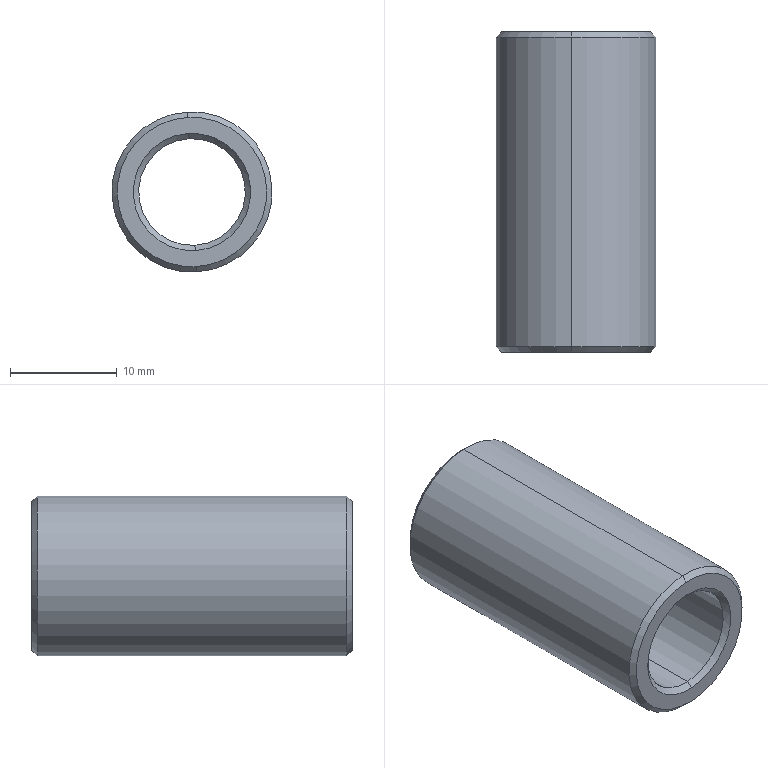Component | SolidWorks | JB_T8013.1-1999LocatingBushingA18-3 | 1 solid | 14 faces | box 15 x 30 x 15 mm | volume 2923 mm3 | cone 6 | cylinder 4 | torus 2 | plane 2 | commonest cylinder face diameters 10 x2 15 x2 | material Nickel
build123d program:
from build123d import *

# Parameters (mm, degrees)
SKETCH1_R          = 7.5
SKETCH1_R_2        = 5
BASE_EXTRUDE_DEPTH = 30
FILLET1_R          = 1
CHAMFER1_SIZE      = 0.5


with BuildPart() as part:
    # Sketch1 → Base-Extrude (new body)
    with BuildSketch(Plane.XY):
        Circle(SKETCH1_R)
        Circle(SKETCH1_R_2, mode=Mode.SUBTRACT)
    extrude(amount=-BASE_EXTRUDE_DEPTH)

    # Fillet1
    fillet1_edges = [part.edges().sort_by_distance(p)[0] for p in [
        (-5, 0, 0),
    ]]
    fillet(fillet1_edges, radius=FILLET1_R)

    # Chamfer1
    chamfer1_edges = [part.edges().sort_by_distance(p)[0] for p in [
        (-7.5, 0, 0),
        (-7.5, 0, -30),
        (-5, 0, -30),
    ]]
    chamfer(chamfer1_edges, length=CHAMFER1_SIZE)


solid = part.part

# Placed as in the assembly
solid = solid.moved(Location((45.466, 305, -26.25), (-90, 0, 0)))
STEP:
#1=COLOUR_RGB('',0.7922,0.8196,0.9333);
#2=FILL_AREA_STYLE_COLOUR('',#1);
#3=FILL_AREA_STYLE('',(#2));
#4=SURFACE_STYLE_FILL_AREA(#3);
#5=SURFACE_SIDE_STYLE('',(#4));
#6=SURFACE_STYLE_USAGE(.BOTH.,#5);
#7=PRESENTATION_STYLE_ASSIGNMENT((#6));
#8=CARTESIAN_POINT('',(1.775,12.008,-0.7583));
#9=VERTEX_POINT('',#8);
#10=CARTESIAN_POINT('',(1.805,12.008,-1.309));
#11=VERTEX_POINT('',#10);
#12=CARTESIAN_POINT('',(1.79,12.008,-1.033));
#13=DIRECTION('',(0.,1.,0.));
#14=DIRECTION('',(-0.05508,0.,0.9985));
#15=AXIS2_PLACEMENT_3D('',#12,#13,#14);
#16=CIRCLE('',#15,0.2756);
#17=EDGE_CURVE('',#9,#11,#16,.T.);
#18=ORIENTED_EDGE('',*,*,#17,.F.);
#19=CARTESIAN_POINT('',(1.774,11.988,-0.7386));
#20=VERTEX_POINT('',#19);
#21=CARTESIAN_POINT('',(1.775,12.008,-0.7583));
#22=DIRECTION('',(-0.03895,-0.7071,0.706));
#23=VECTOR('',#22,39.37);
#24=LINE('',#21,#23);
#25=EDGE_CURVE('',#9,#20,#24,.T.);
#26=ORIENTED_EDGE('',*,*,#25,.T.);
#27=CARTESIAN_POINT('',(1.806,11.988,-1.328));
#28=VERTEX_POINT('',#27);
#29=CARTESIAN_POINT('',(1.79,11.988,-1.033));
#30=DIRECTION('',(0.,-1.,0.));
#31=DIRECTION('',(-0.05508,0.,0.9985));
#32=AXIS2_PLACEMENT_3D('',#29,#30,#31);
#33=CIRCLE('',#32,0.2953);
#34=EDGE_CURVE('',#28,#20,#33,.T.);
#35=ORIENTED_EDGE('',*,*,#34,.F.);
#36=CARTESIAN_POINT('',(1.805,12.008,-1.309));
#37=DIRECTION('',(0.03895,-0.7071,-0.706));
#38=VECTOR('',#37,39.37);
#39=LINE('',#36,#38);
#40=EDGE_CURVE('',#11,#28,#39,.T.);
#41=ORIENTED_EDGE('',*,*,#40,.F.);
#42=EDGE_LOOP('',(#18,#26,#35,#41));
#43=FACE_OUTER_BOUND('',#42,.T.);
#44=CARTESIAN_POINT('',(1.79,12.008,-1.033));
#45=DIRECTION('',(0.,-1.,0.));
#46=DIRECTION('',(0.05508,0.,-0.9985));
#47=AXIS2_PLACEMENT_3D('',#44,#45,#46);
#48=CONICAL_SURFACE('',#47,0.2756,0.7854);
#49=ADVANCED_FACE('',(#43),#48,.T.);
#50=CARTESIAN_POINT('',(1.805,10.827,-1.309));
#51=VERTEX_POINT('',#50);
#52=CARTESIAN_POINT('',(1.775,10.827,-0.7583));
#53=VERTEX_POINT('',#52);
#54=CARTESIAN_POINT('',(1.79,10.827,-1.033));
#55=DIRECTION('',(0.,-1.,0.));
#56=DIRECTION('',(-0.05508,0.,0.9985));
#57=AXIS2_PLACEMENT_3D('',#54,#55,#56);
#58=CIRCLE('',#57,0.2756);
#59=EDGE_CURVE('',#51,#53,#58,.T.);
#60=ORIENTED_EDGE('',*,*,#59,.F.);
#61=CARTESIAN_POINT('',(1.806,10.846,-1.328));
#62=VERTEX_POINT('',#61);
#63=CARTESIAN_POINT('',(1.806,10.846,-1.328));
#64=DIRECTION('',(0.03895,0.7071,-0.706));
#65=VECTOR('',#64,39.37);
#66=LINE('',#63,#65);
#67=EDGE_CURVE('',#51,#62,#66,.T.);
#68=ORIENTED_EDGE('',*,*,#67,.T.);
#69=CARTESIAN_POINT('',(1.774,10.846,-0.7386));
#70=VERTEX_POINT('',#69);
#71=CARTESIAN_POINT('',(1.79,10.846,-1.033));
#72=DIRECTION('',(0.,1.,0.));
#73=DIRECTION('',(-0.05508,0.,0.9985));
#74=AXIS2_PLACEMENT_3D('',#71,#72,#73);
#75=CIRCLE('',#74,0.2953);
#76=EDGE_CURVE('',#70,#62,#75,.T.);
#77=ORIENTED_EDGE('',*,*,#76,.F.);
#78=CARTESIAN_POINT('',(1.774,10.846,-0.7386));
#79=DIRECTION('',(-0.03895,0.7071,0.706));
#80=VECTOR('',#79,39.37);
#81=LINE('',#78,#80);
#82=EDGE_CURVE('',#53,#70,#81,.T.);
#83=ORIENTED_EDGE('',*,*,#82,.F.);
#84=EDGE_LOOP('',(#60,#68,#77,#83));
#85=FACE_OUTER_BOUND('',#84,.T.);
#86=CARTESIAN_POINT('',(1.79,10.846,-1.033));
#87=DIRECTION('',(0.,1.,0.));
#88=DIRECTION('',(-0.05508,0.,0.9985));
#89=AXIS2_PLACEMENT_3D('',#86,#87,#88);
#90=CONICAL_SURFACE('',#89,0.2953,0.7854);
#91=ADVANCED_FACE('',(#85),#90,.T.);
#92=CARTESIAN_POINT('',(1.779,10.846,-0.8369));
#93=VERTEX_POINT('',#92);
#94=CARTESIAN_POINT('',(1.801,10.846,-1.23));
#95=VERTEX_POINT('',#94);
#96=CARTESIAN_POINT('',(1.79,10.846,-1.033));
#97=DIRECTION('',(0.,-1.,0.));
#98=DIRECTION('',(-0.05508,0.,0.9985));
#99=AXIS2_PLACEMENT_3D('',#96,#97,#98);
#100=CIRCLE('',#99,0.1969);
#101=EDGE_CURVE('',#93,#95,#100,.T.);
#102=ORIENTED_EDGE('',*,*,#101,.F.);
#103=CARTESIAN_POINT('',(1.778,10.827,-0.8173));
#104=VERTEX_POINT('',#103);
#105=CARTESIAN_POINT('',(1.778,10.827,-0.8173));
#106=DIRECTION('',(-0.03895,-0.7071,0.706));
#107=VECTOR('',#106,39.37);
#108=LINE('',#105,#107);
#109=EDGE_CURVE('',#93,#104,#108,.T.);
#110=ORIENTED_EDGE('',*,*,#109,.T.);
#111=CARTESIAN_POINT('',(1.802,10.827,-1.25));
#112=VERTEX_POINT('',#111);
#113=CARTESIAN_POINT('',(1.79,10.827,-1.033));
#114=DIRECTION('',(0.,1.,0.));
#115=DIRECTION('',(-0.05508,0.,0.9985));
#116=AXIS2_PLACEMENT_3D('',#113,#114,#115);
#117=CIRCLE('',#116,0.2165);
#118=EDGE_CURVE('',#112,#104,#117,.T.);
#119=ORIENTED_EDGE('',*,*,#118,.F.);
#120=CARTESIAN_POINT('',(1.802,10.827,-1.25));
#121=DIRECTION('',(0.03895,-0.7071,-0.706));
#122=VECTOR('',#121,39.37);
#123=LINE('',#120,#122);
#124=EDGE_CURVE('',#95,#112,#123,.T.);
#125=ORIENTED_EDGE('',*,*,#124,.F.);
#126=EDGE_LOOP('',(#102,#110,#119,#125));
#127=FACE_OUTER_BOUND('',#126,.T.);
#128=CARTESIAN_POINT('',(1.79,10.827,-1.033));
#129=DIRECTION('',(0.,-1.,0.));
#130=DIRECTION('',(0.05508,0.,-0.9985));
#131=AXIS2_PLACEMENT_3D('',#128,#129,#130);
#132=CONICAL_SURFACE('',#131,0.2165,0.7854);
#133=ADVANCED_FACE('',(#127),#132,.F.);
#134=CARTESIAN_POINT('',(1.803,12.008,-1.269));
#135=VERTEX_POINT('',#134);
#136=CARTESIAN_POINT('',(1.777,12.008,-0.7976));
#137=VERTEX_POINT('',#136);
#138=CARTESIAN_POINT('',(1.79,12.008,-1.033));
#139=DIRECTION('',(0.,-1.,0.));
#140=DIRECTION('',(-0.05508,0.,0.9985));
#141=AXIS2_PLACEMENT_3D('',#138,#139,#140);
#142=CIRCLE('',#141,0.2362);
#143=EDGE_CURVE('',#135,#137,#142,.T.);
#144=ORIENTED_EDGE('',*,*,#143,.F.);
#145=CARTESIAN_POINT('',(1.801,11.969,-1.23));
#146=VERTEX_POINT('',#145);
#147=CARTESIAN_POINT('',(1.803,11.969,-1.269));
#148=DIRECTION('',(0.9985,0.,0.05508));
#149=DIRECTION('',(0.05508,0.,-0.9985));
#150=AXIS2_PLACEMENT_3D('',#147,#148,#149);
#151=CIRCLE('',#150,0.03937);
#152=EDGE_CURVE('',#135,#146,#151,.T.);
#153=ORIENTED_EDGE('',*,*,#152,.T.);
#154=CARTESIAN_POINT('',(1.779,11.969,-0.8369));
#155=VERTEX_POINT('',#154);
#156=CARTESIAN_POINT('',(1.79,11.969,-1.033));
#157=DIRECTION('',(0.,1.,0.));
#158=DIRECTION('',(-0.05508,0.,0.9985));
#159=AXIS2_PLACEMENT_3D('',#156,#157,#158);
#160=CIRCLE('',#159,0.1969);
#161=EDGE_CURVE('',#155,#146,#160,.T.);
#162=ORIENTED_EDGE('',*,*,#161,.F.);
#163=CARTESIAN_POINT('',(1.777,11.969,-0.7976));
#164=DIRECTION('',(-0.9985,0.,-0.05508));
#165=DIRECTION('',(-0.05508,0.,0.9985));
#166=AXIS2_PLACEMENT_3D('',#163,#164,#165);
#167=CIRCLE('',#166,0.03937);
#168=EDGE_CURVE('',#137,#155,#167,.T.);
#169=ORIENTED_EDGE('',*,*,#168,.F.);
#170=EDGE_LOOP('',(#144,#153,#162,#169));
#171=FACE_OUTER_BOUND('',#170,.T.);
#172=CARTESIAN_POINT('',(1.79,11.969,-1.033));
#173=DIRECTION('',(0.,1.,0.));
#174=DIRECTION('',(-0.05508,0.,0.9985));
#175=AXIS2_PLACEMENT_3D('',#172,#173,#174);
#176=TOROIDAL_SURFACE('',#175,0.2362,0.03937);
#177=ADVANCED_FACE('',(#171),#176,.T.);
#178=ORIENTED_EDGE('',*,*,#101,.T.);
#179=CARTESIAN_POINT('',(1.801,10.827,-1.23));
#180=DIRECTION('',(0.,1.,0.));
#181=VECTOR('',#180,39.37);
#182=LINE('',#179,#181);
#183=EDGE_CURVE('',#95,#146,#182,.T.);
#184=ORIENTED_EDGE('',*,*,#183,.T.);
#185=CARTESIAN_POINT('',(1.79,11.969,-1.033));
#186=DIRECTION('',(0.,1.,0.));
#187=DIRECTION('',(-0.05508,0.,0.9985));
#188=AXIS2_PLACEMENT_3D('',#185,#186,#187);
#189=CIRCLE('',#188,0.1969);
#190=EDGE_CURVE('',#146,#155,#189,.T.);
#191=ORIENTED_EDGE('',*,*,#190,.T.);
#192=CARTESIAN_POINT('',(1.779,10.827,-0.8369));
#193=DIRECTION('',(0.,1.,0.));
#194=VECTOR('',#193,39.37);
#195=LINE('',#192,#194);
#196=EDGE_CURVE('',#93,#155,#195,.T.);
#197=ORIENTED_EDGE('',*,*,#196,.F.);
#198=EDGE_LOOP('',(#178,#184,#191,#197));
#199=FACE_OUTER_BOUND('',#198,.T.);
#200=CARTESIAN_POINT('',(1.79,10.827,-1.033));
#201=DIRECTION('',(0.,1.,0.));
#202=DIRECTION('',(-0.05508,0.,0.9985));
#203=AXIS2_PLACEMENT_3D('',#200,#201,#202);
#204=CYLINDRICAL_SURFACE('',#203,0.1969);
#205=ADVANCED_FACE('',(#199),#204,.F.);
#206=ORIENTED_EDGE('',*,*,#76,.T.);
#207=CARTESIAN_POINT('',(1.806,10.827,-1.328));
#208=DIRECTION('',(0.,1.,0.));
#209=VECTOR('',#208,39.37);
#210=LINE('',#207,#209);
#211=EDGE_CURVE('',#62,#28,#210,.T.);
#212=ORIENTED_EDGE('',*,*,#211,.T.);
#213=ORIENTED_EDGE('',*,*,#34,.T.);
#214=CARTESIAN_POINT('',(1.774,10.827,-0.7386));
#215=DIRECTION('',(0.,1.,0.));
#216=VECTOR('',#215,39.37);
#217=LINE('',#214,#216);
#218=EDGE_CURVE('',#70,#20,#217,.T.);
#219=ORIENTED_EDGE('',*,*,#218,.F.);
#220=EDGE_LOOP('',(#206,#212,#213,#219));
#221=FACE_OUTER_BOUND('',#220,.T.);
#222=CARTESIAN_POINT('',(1.79,10.827,-1.033));
#223=DIRECTION('',(0.,1.,0.));
#224=DIRECTION('',(-0.05508,0.,0.9985));
#225=AXIS2_PLACEMENT_3D('',#222,#223,#224);
#226=CYLINDRICAL_SURFACE('',#225,0.2953);
#227=ADVANCED_FACE('',(#221),#226,.T.);
#228=ORIENTED_EDGE('',*,*,#211,.F.);
#229=CARTESIAN_POINT('',(1.79,10.846,-1.033));
#230=DIRECTION('',(0.,1.,0.));
#231=DIRECTION('',(-0.05508,0.,0.9985));
#232=AXIS2_PLACEMENT_3D('',#229,#230,#231);
#233=CIRCLE('',#232,0.2953);
#234=EDGE_CURVE('',#62,#70,#233,.T.);
#235=ORIENTED_EDGE('',*,*,#234,.T.);
#236=ORIENTED_EDGE('',*,*,#218,.T.);
#237=CARTESIAN_POINT('',(1.79,11.988,-1.033));
#238=DIRECTION('',(0.,-1.,0.));
#239=DIRECTION('',(-0.05508,0.,0.9985));
#240=AXIS2_PLACEMENT_3D('',#237,#238,#239);
#241=CIRCLE('',#240,0.2953);
#242=EDGE_CURVE('',#20,#28,#241,.T.);
#243=ORIENTED_EDGE('',*,*,#242,.T.);
#244=EDGE_LOOP('',(#228,#235,#236,#243));
#245=FACE_OUTER_BOUND('',#244,.T.);
#246=CARTESIAN_POINT('',(1.79,10.827,-1.033));
#247=DIRECTION('',(0.,1.,0.));
#248=DIRECTION('',(-0.05508,0.,0.9985));
#249=AXIS2_PLACEMENT_3D('',#246,#247,#248);
#250=CYLINDRICAL_SURFACE('',#249,0.2953);
#251=ADVANCED_FACE('',(#245),#250,.T.);
#252=ORIENTED_EDGE('',*,*,#118,.T.);
#253=CARTESIAN_POINT('',(1.79,10.827,-1.033));
#254=DIRECTION('',(0.,1.,0.));
#255=DIRECTION('',(-0.05508,0.,0.9985));
#256=AXIS2_PLACEMENT_3D('',#253,#254,#255);
#257=CIRCLE('',#256,0.2165);
#258=EDGE_CURVE('',#104,#112,#257,.T.);
#259=ORIENTED_EDGE('',*,*,#258,.T.);
#260=EDGE_LOOP('',(#252,#259));
#261=FACE_BOUND('',#260,.T.);
#262=CARTESIAN_POINT('',(1.79,10.827,-1.033));
#263=DIRECTION('',(0.,-1.,0.));
#264=DIRECTION('',(-0.05508,0.,0.9985));
#265=AXIS2_PLACEMENT_3D('',#262,#263,#264);
#266=CIRCLE('',#265,0.2756);
#267=EDGE_CURVE('',#53,#51,#266,.T.);
#268=ORIENTED_EDGE('',*,*,#267,.T.);
#269=ORIENTED_EDGE('',*,*,#59,.T.);
#270=EDGE_LOOP('',(#268,#269));
#271=FACE_OUTER_BOUND('',#270,.T.);
#272=CARTESIAN_POINT('',(1.79,10.827,-1.033));
#273=DIRECTION('',(0.,1.,0.));
#274=DIRECTION('',(-0.05508,0.,0.9985));
#275=AXIS2_PLACEMENT_3D('',#272,#273,#274);
#276=PLANE('',#275);
#277=ADVANCED_FACE('',(#261,#271),#276,.F.);
#278=CARTESIAN_POINT('',(1.79,12.008,-1.033));
#279=DIRECTION('',(0.,1.,0.));
#280=DIRECTION('',(-0.05508,0.,0.9985));
#281=AXIS2_PLACEMENT_3D('',#278,#279,#280);
#282=CIRCLE('',#281,0.2756);
#283=EDGE_CURVE('',#11,#9,#282,.T.);
#284=ORIENTED_EDGE('',*,*,#283,.T.);
#285=ORIENTED_EDGE('',*,*,#17,.T.);
#286=EDGE_LOOP('',(#284,#285));
#287=FACE_OUTER_BOUND('',#286,.T.);
#288=CARTESIAN_POINT('',(1.79,12.008,-1.033));
#289=DIRECTION('',(0.,-1.,0.));
#290=DIRECTION('',(-0.05508,0.,0.9985));
#291=AXIS2_PLACEMENT_3D('',#288,#289,#290);
#292=CIRCLE('',#291,0.2362);
#293=EDGE_CURVE('',#137,#135,#292,.T.);
#294=ORIENTED_EDGE('',*,*,#293,.T.);
#295=ORIENTED_EDGE('',*,*,#143,.T.);
#296=EDGE_LOOP('',(#294,#295));
#297=FACE_BOUND('',#296,.T.);
#298=CARTESIAN_POINT('',(1.79,12.008,-1.033));
#299=DIRECTION('',(0.,1.,0.));
#300=DIRECTION('',(-0.05508,0.,0.9985));
#301=AXIS2_PLACEMENT_3D('',#298,#299,#300);
#302=PLANE('',#301);
#303=ADVANCED_FACE('',(#287,#297),#302,.T.);
#304=ORIENTED_EDGE('',*,*,#183,.F.);
#305=CARTESIAN_POINT('',(1.79,10.846,-1.033));
#306=DIRECTION('',(0.,-1.,0.));
#307=DIRECTION('',(-0.05508,0.,0.9985));
#308=AXIS2_PLACEMENT_3D('',#305,#306,#307);
#309=CIRCLE('',#308,0.1969);
#310=EDGE_CURVE('',#95,#93,#309,.T.);
#311=ORIENTED_EDGE('',*,*,#310,.T.);
#312=ORIENTED_EDGE('',*,*,#196,.T.);
#313=ORIENTED_EDGE('',*,*,#161,.T.);
#314=EDGE_LOOP('',(#304,#311,#312,#313));
#315=FACE_OUTER_BOUND('',#314,.T.);
#316=CARTESIAN_POINT('',(1.79,10.827,-1.033));
#317=DIRECTION('',(0.,1.,0.));
#318=DIRECTION('',(-0.05508,0.,0.9985));
#319=AXIS2_PLACEMENT_3D('',#316,#317,#318);
#320=CYLINDRICAL_SURFACE('',#319,0.1969);
#321=ADVANCED_FACE('',(#315),#320,.F.);
#322=ORIENTED_EDGE('',*,*,#152,.F.);
#323=ORIENTED_EDGE('',*,*,#293,.F.);
#324=ORIENTED_EDGE('',*,*,#168,.T.);
#325=ORIENTED_EDGE('',*,*,#190,.F.);
#326=EDGE_LOOP('',(#322,#323,#324,#325));
#327=FACE_OUTER_BOUND('',#326,.T.);
#328=CARTESIAN_POINT('',(1.79,11.969,-1.033));
#329=DIRECTION('',(0.,1.,0.));
#330=DIRECTION('',(-0.05508,0.,0.9985));
#331=AXIS2_PLACEMENT_3D('',#328,#329,#330);
#332=TOROIDAL_SURFACE('',#331,0.2362,0.03937);
#333=ADVANCED_FACE('',(#327),#332,.T.);
#334=ORIENTED_EDGE('',*,*,#109,.F.);
#335=ORIENTED_EDGE('',*,*,#310,.F.);
#336=ORIENTED_EDGE('',*,*,#124,.T.);
#337=ORIENTED_EDGE('',*,*,#258,.F.);
#338=EDGE_LOOP('',(#334,#335,#336,#337));
#339=FACE_OUTER_BOUND('',#338,.T.);
#340=CARTESIAN_POINT('',(1.79,10.827,-1.033));
#341=DIRECTION('',(0.,-1.,0.));
#342=DIRECTION('',(0.05508,0.,-0.9985));
#343=AXIS2_PLACEMENT_3D('',#340,#341,#342);
#344=CONICAL_SURFACE('',#343,0.2165,0.7854);
#345=ADVANCED_FACE('',(#339),#344,.F.);
#346=ORIENTED_EDGE('',*,*,#67,.F.);
#347=ORIENTED_EDGE('',*,*,#267,.F.);
#348=ORIENTED_EDGE('',*,*,#82,.T.);
#349=ORIENTED_EDGE('',*,*,#234,.F.);
#350=EDGE_LOOP('',(#346,#347,#348,#349));
#351=FACE_OUTER_BOUND('',#350,.T.);
#352=CARTESIAN_POINT('',(1.79,10.846,-1.033));
#353=DIRECTION('',(0.,1.,0.));
#354=DIRECTION('',(-0.05508,0.,0.9985));
#355=AXIS2_PLACEMENT_3D('',#352,#353,#354);
#356=CONICAL_SURFACE('',#355,0.2953,0.7854);
#357=ADVANCED_FACE('',(#351),#356,.T.);
#358=ORIENTED_EDGE('',*,*,#25,.F.);
#359=ORIENTED_EDGE('',*,*,#283,.F.);
#360=ORIENTED_EDGE('',*,*,#40,.T.);
#361=ORIENTED_EDGE('',*,*,#242,.F.);
#362=EDGE_LOOP('',(#358,#359,#360,#361));
#363=FACE_OUTER_BOUND('',#362,.T.);
#364=CARTESIAN_POINT('',(1.79,12.008,-1.033));
#365=DIRECTION('',(0.,-1.,0.));
#366=DIRECTION('',(0.05508,0.,-0.9985));
#367=AXIS2_PLACEMENT_3D('',#364,#365,#366);
#368=CONICAL_SURFACE('',#367,0.2756,0.7854);
#369=ADVANCED_FACE('',(#363),#368,.T.);
#370=CLOSED_SHELL('',(#49,#91,#133,#177,#205,#227,#251,#277,#303,#321,#333,#345,#357,#369));
#371=MANIFOLD_SOLID_BREP('',#370);
#372=STYLED_ITEM('',(#7),#371);
#373=PRESENTATION_LAYER_ASSIGNMENT('','',(#372));
#374=CARTESIAN_POINT('',(0.,0.,0.));
#375=DIRECTION('',(0.,0.,1.));
#376=DIRECTION('',(1.,0.,0.));
#377=AXIS2_PLACEMENT_3D('',#374,#375,#376);
#378=(LENGTH_UNIT()NAMED_UNIT(*)SI_UNIT($,.METRE.));
#379=LENGTH_MEASURE_WITH_UNIT(LENGTH_MEASURE(0.0254),#378);
#380=DIMENSIONAL_EXPONENTS(1.,0.,0.,0.,0.,0.,0.);
#381=(CONVERSION_BASED_UNIT('',#379)LENGTH_UNIT()NAMED_UNIT(#380));
#382=UNCERTAINTY_MEASURE_WITH_UNIT(LENGTH_MEASURE(0.00001),#381,'','');
#383=(NAMED_UNIT(*)PLANE_ANGLE_UNIT()SI_UNIT($,.RADIAN.));
#384=(NAMED_UNIT(*)SI_UNIT($,.STERADIAN.)SOLID_ANGLE_UNIT());
#385=(GEOMETRIC_REPRESENTATION_CONTEXT(3)GLOBAL_UNCERTAINTY_ASSIGNED_CONTEXT((#382))GLOBAL_UNIT_ASSIGNED_CONTEXT((#381,#383,#384))REPRESENTATION_CONTEXT('',''));
#386=ADVANCED_BREP_SHAPE_REPRESENTATION('',(#371,#377),#385);
#387=(LENGTH_UNIT()NAMED_UNIT(*)SI_UNIT($,.METRE.));
#388=LENGTH_MEASURE_WITH_UNIT(LENGTH_MEASURE(0.0254),#387);
#389=DIMENSIONAL_EXPONENTS(1.,0.,0.,0.,0.,0.,0.);
#390=(CONVERSION_BASED_UNIT('',#388)LENGTH_UNIT()NAMED_UNIT(#389));
#391=UNCERTAINTY_MEASURE_WITH_UNIT(LENGTH_MEASURE(0.00001),#390,'','');
#392=(NAMED_UNIT(*)PLANE_ANGLE_UNIT()SI_UNIT($,.RADIAN.));
#393=(NAMED_UNIT(*)SI_UNIT($,.STERADIAN.)SOLID_ANGLE_UNIT());
#394=(GEOMETRIC_REPRESENTATION_CONTEXT(3)GLOBAL_UNCERTAINTY_ASSIGNED_CONTEXT((#391))GLOBAL_UNIT_ASSIGNED_CONTEXT((#390,#392,#393))REPRESENTATION_CONTEXT('',''));
#395=MECHANICAL_DESIGN_GEOMETRIC_PRESENTATION_REPRESENTATION('',(#372),#394);